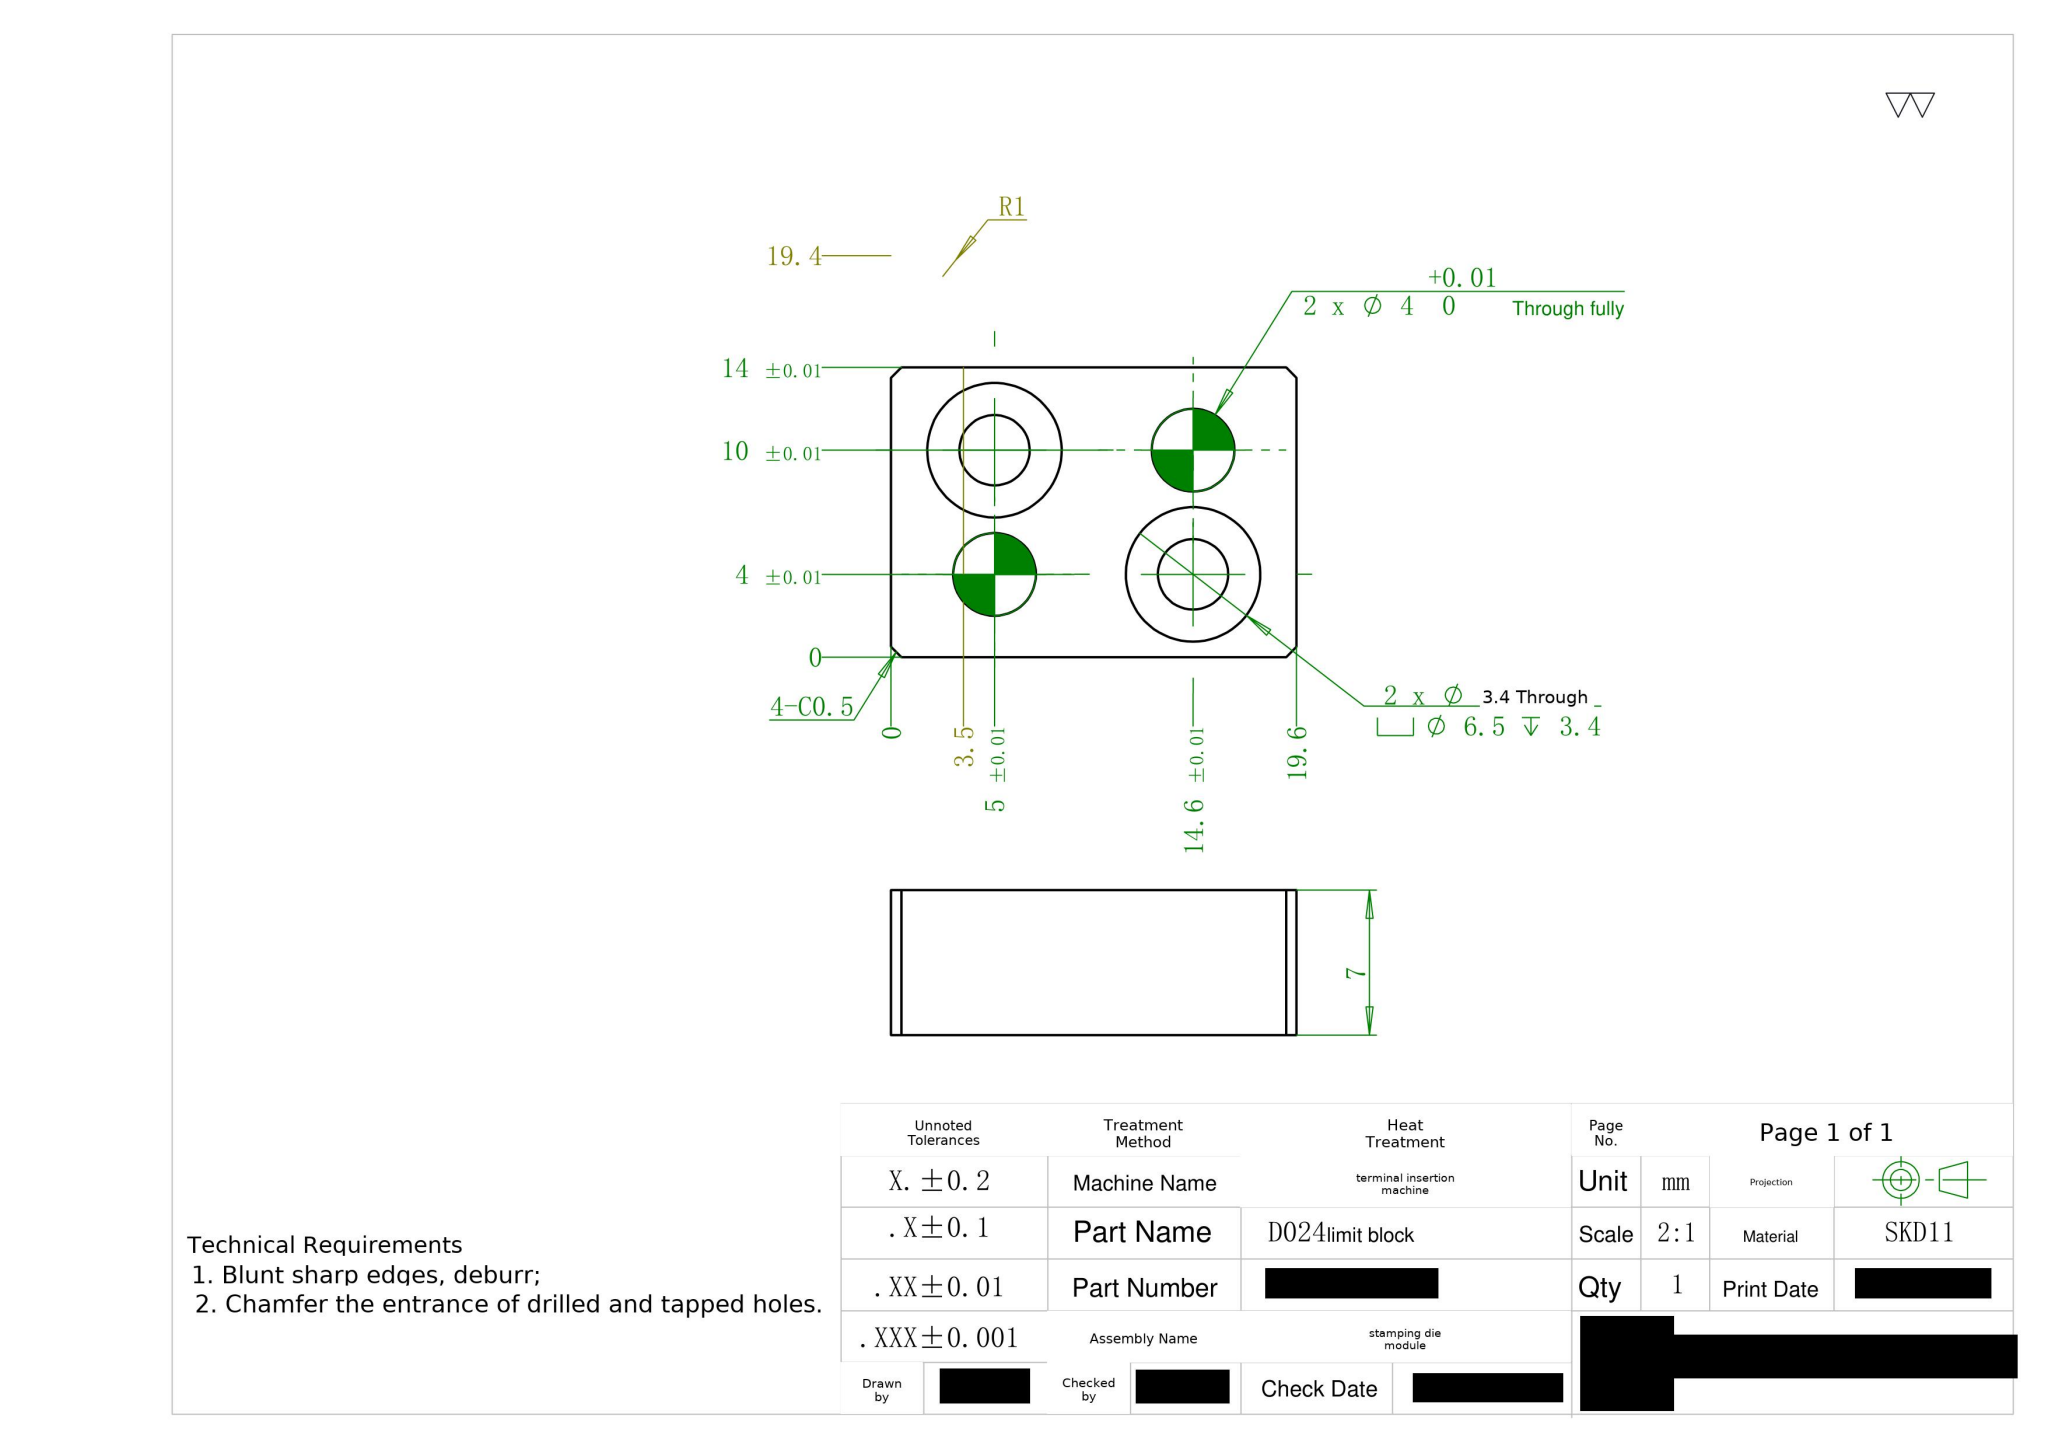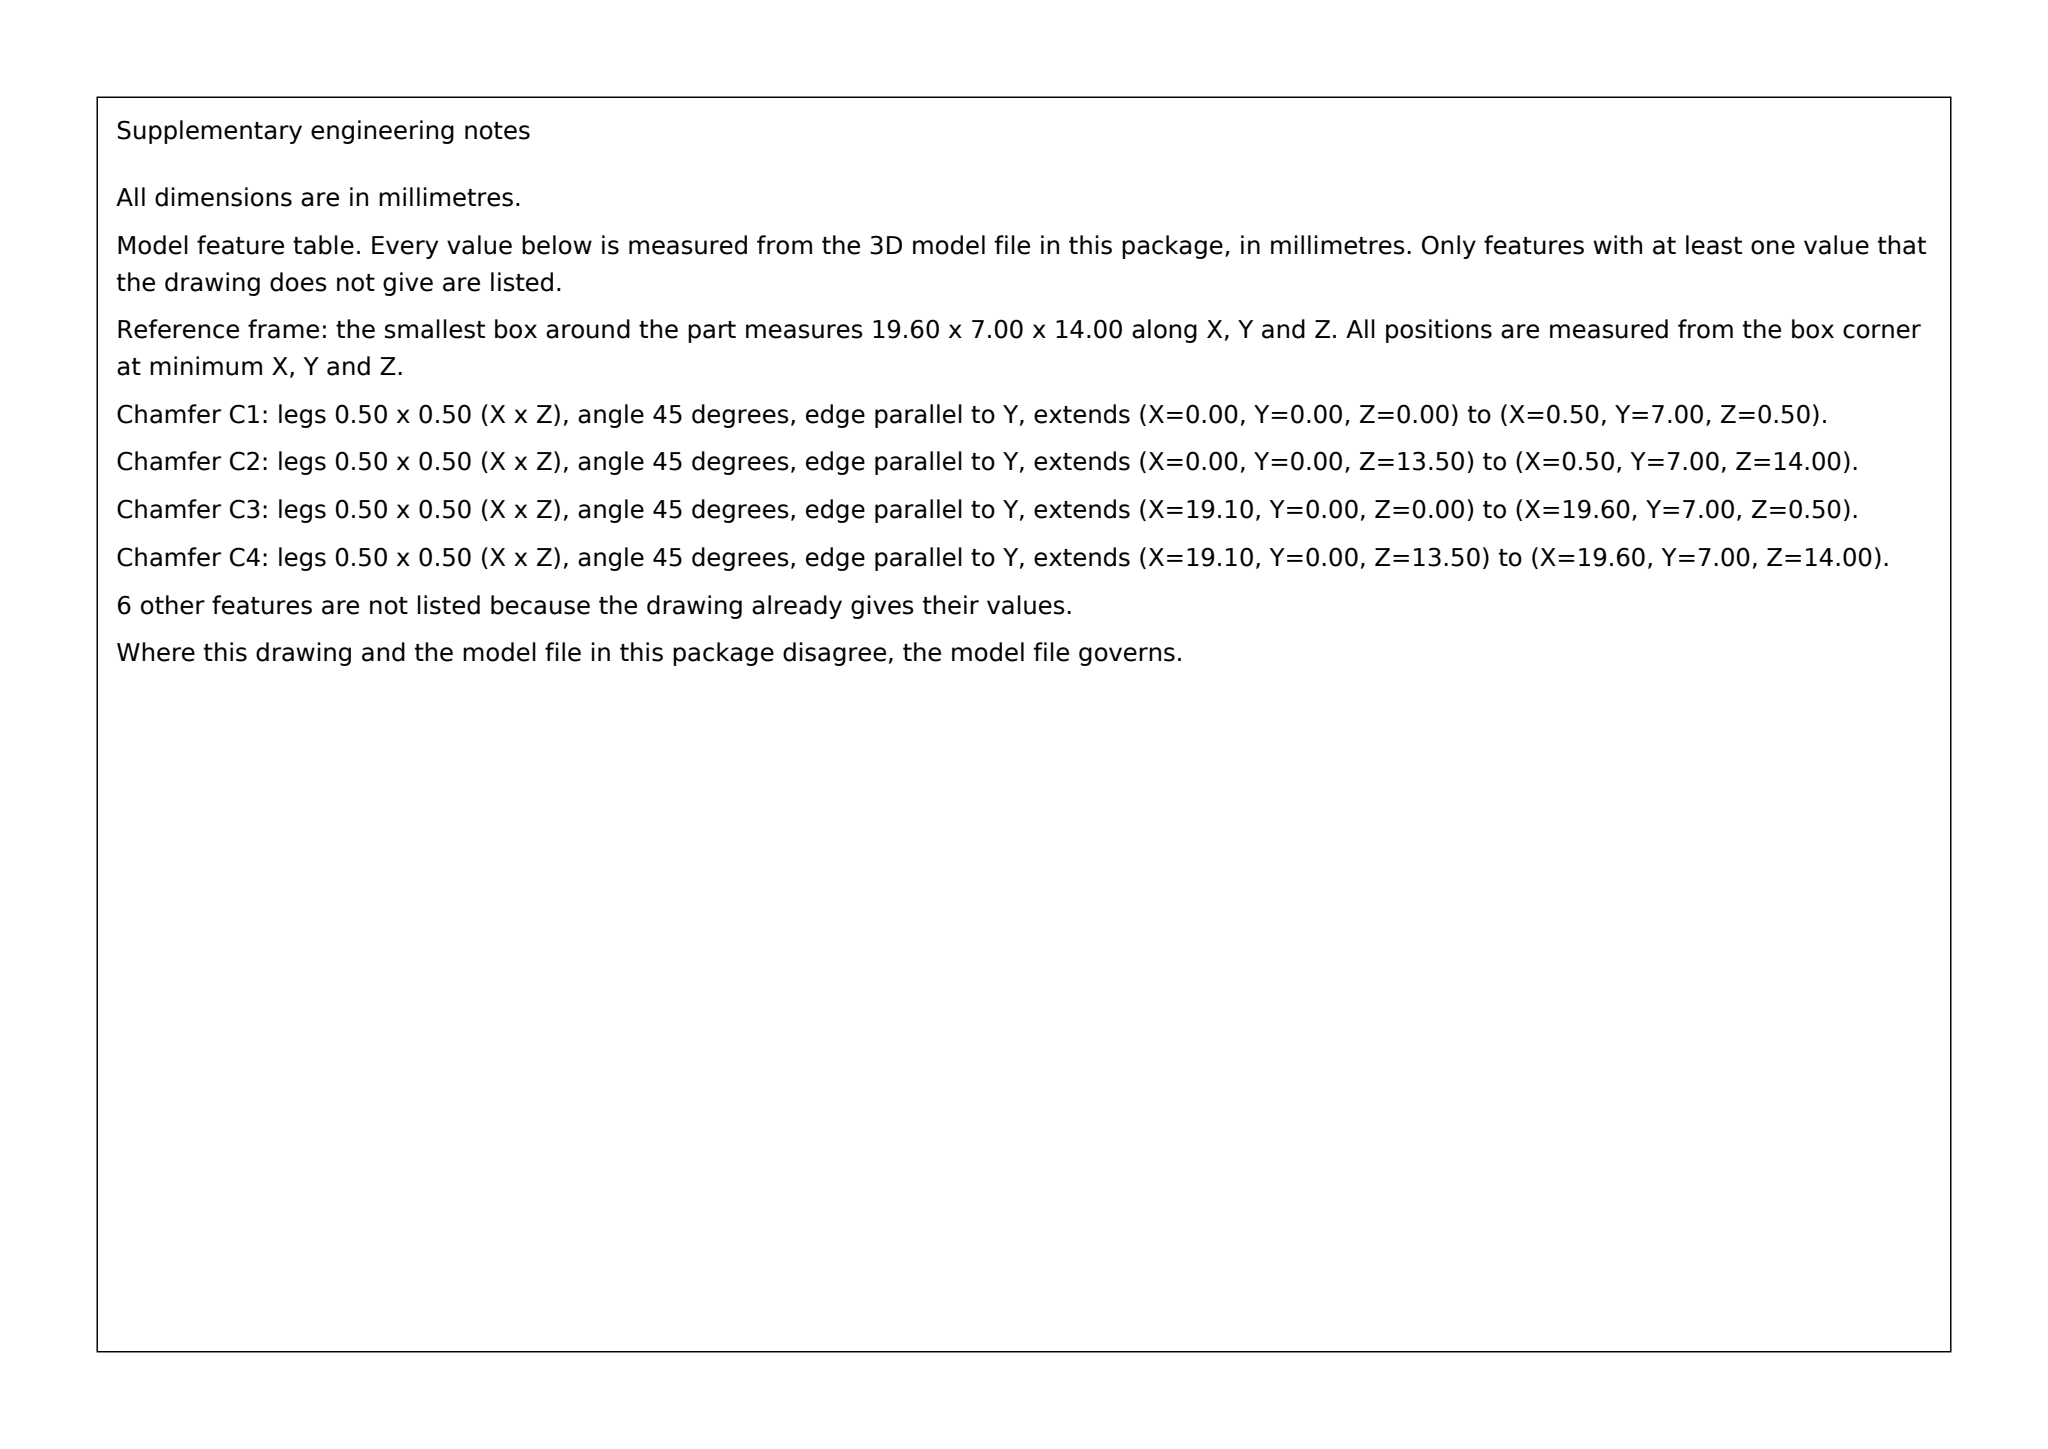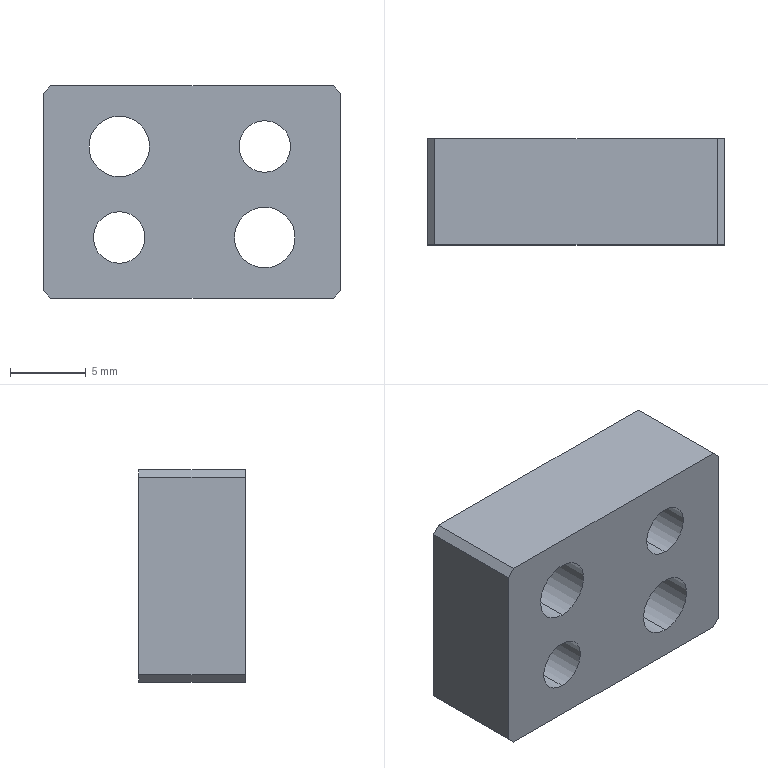Part | SolidWorks | mm | 1 solid | 24 faces | box 19.6 x 7 x 14 mm | volume 1450 mm3 | cylinder 12 | plane 12 | commonest cylinder face diameters 4 x4 6.5 x4 3.4 x4
build123d program:
from build123d import *

# Parameters (mm, degrees)
SKETCH1_W                                       = 19.6
SKETCH1_H                                       = 14
BOSS_EXTRUDE1_DEPTH                             = 7
M3_HEX_SOCKET_HEAD_CAP_SCREW_CBORE1_D           = 3.4
M3_HEX_SOCKET_HEAD_CAP_SCREW_CBORE1_CBORE_D     = 6.5
M3_HEX_SOCKET_HEAD_CAP_SCREW_CBORE1_CBORE_DEPTH = 3.4
F_4_0_4_DIAMETER_HOLE1_D                        = 4
CHAMFER1_SIZE                                   = 0.5


with BuildPart() as part:
    # Sketch1 → Boss-Extrude1 (new body)
    with BuildSketch(Plane(origin=(0, 0, 0), x_dir=(1, 0, 0), z_dir=(0, 1, 0))):
        Rectangle(SKETCH1_W, SKETCH1_H)
    extrude(amount=BOSS_EXTRUDE1_DEPTH)

    # M3 Hex Socket Head Cap Screw CBORE1 (through all)
    with Locations(Plane(origin=(0, 7, 0), x_dir=(1, 0, 0), z_dir=(0, 1, 0))):
        with Locations((4.8, -3), (-4.8, 3)):
            CounterBoreHole(M3_HEX_SOCKET_HEAD_CAP_SCREW_CBORE1_D / 2, M3_HEX_SOCKET_HEAD_CAP_SCREW_CBORE1_CBORE_D / 2, M3_HEX_SOCKET_HEAD_CAP_SCREW_CBORE1_CBORE_DEPTH)

    # 4.0 _4_ Diameter Hole1 (through all)
    with Locations(Plane(origin=(0, 7, 0), x_dir=(1, 0, 0), z_dir=(0, 1, 0))):
        with Locations((4.8, 3), (-4.8, -3)):
            Hole(F_4_0_4_DIAMETER_HOLE1_D / 2)

    # Chamfer1
    chamfer1_edges = [part.edges().sort_by_distance(p)[0] for p in [
        (9.8, 3.5, 7),
        (-9.8, 3.5, 7),
        (-9.8, 3.5, -7),
        (9.8, 3.5, -7),
    ]]
    chamfer(chamfer1_edges, length=CHAMFER1_SIZE)


solid = part.part
STEP:
#1=CARTESIAN_POINT('',(4.8,0.,-5.));
#2=VERTEX_POINT('',#1);
#3=CARTESIAN_POINT('',(4.8,0.,-1.));
#4=VERTEX_POINT('',#3);
#5=CARTESIAN_POINT('',(4.8,0.,-3.));
#6=DIRECTION('',(0.,1.,0.));
#7=DIRECTION('',(0.,0.,1.));
#8=AXIS2_PLACEMENT_3D('',#5,#6,#7);
#9=CIRCLE('',#8,2.);
#10=EDGE_CURVE('',#2,#4,#9,.T.);
#11=ORIENTED_EDGE('',*,*,#10,.F.);
#12=CARTESIAN_POINT('',(4.8,7.,-5.));
#13=VERTEX_POINT('',#12);
#14=CARTESIAN_POINT('',(4.8,7.,-5.));
#15=DIRECTION('',(0.,1.,0.));
#16=VECTOR('',#15,1000.);
#17=LINE('',#14,#16);
#18=EDGE_CURVE('',#2,#13,#17,.T.);
#19=ORIENTED_EDGE('',*,*,#18,.T.);
#20=CARTESIAN_POINT('',(4.8,7.,-1.));
#21=VERTEX_POINT('',#20);
#22=CARTESIAN_POINT('',(4.8,7.,-3.));
#23=DIRECTION('',(0.,1.,0.));
#24=DIRECTION('',(0.,0.,1.));
#25=AXIS2_PLACEMENT_3D('',#22,#23,#24);
#26=CIRCLE('',#25,2.);
#27=EDGE_CURVE('',#13,#21,#26,.T.);
#28=ORIENTED_EDGE('',*,*,#27,.T.);
#29=CARTESIAN_POINT('',(4.8,7.,-1.));
#30=DIRECTION('',(0.,1.,0.));
#31=VECTOR('',#30,1000.);
#32=LINE('',#29,#31);
#33=EDGE_CURVE('',#4,#21,#32,.T.);
#34=ORIENTED_EDGE('',*,*,#33,.F.);
#35=EDGE_LOOP('',(#11,#19,#28,#34));
#36=FACE_OUTER_BOUND('',#35,.T.);
#37=CARTESIAN_POINT('',(4.8,7.,-3.));
#38=DIRECTION('',(0.,1.,0.));
#39=DIRECTION('',(0.,0.,1.));
#40=AXIS2_PLACEMENT_3D('',#37,#38,#39);
#41=CYLINDRICAL_SURFACE('',#40,2.);
#42=ADVANCED_FACE('',(#36),#41,.F.);
#43=CARTESIAN_POINT('',(-4.8,0.,1.));
#44=VERTEX_POINT('',#43);
#45=CARTESIAN_POINT('',(-4.8,0.,5.));
#46=VERTEX_POINT('',#45);
#47=CARTESIAN_POINT('',(-4.8,0.,3.));
#48=DIRECTION('',(0.,1.,0.));
#49=DIRECTION('',(0.,0.,1.));
#50=AXIS2_PLACEMENT_3D('',#47,#48,#49);
#51=CIRCLE('',#50,2.);
#52=EDGE_CURVE('',#44,#46,#51,.T.);
#53=ORIENTED_EDGE('',*,*,#52,.F.);
#54=CARTESIAN_POINT('',(-4.8,7.,1.));
#55=VERTEX_POINT('',#54);
#56=CARTESIAN_POINT('',(-4.8,7.,1.));
#57=DIRECTION('',(0.,1.,0.));
#58=VECTOR('',#57,1000.);
#59=LINE('',#56,#58);
#60=EDGE_CURVE('',#44,#55,#59,.T.);
#61=ORIENTED_EDGE('',*,*,#60,.T.);
#62=CARTESIAN_POINT('',(-4.8,7.,5.));
#63=VERTEX_POINT('',#62);
#64=CARTESIAN_POINT('',(-4.8,7.,3.));
#65=DIRECTION('',(0.,1.,0.));
#66=DIRECTION('',(0.,0.,1.));
#67=AXIS2_PLACEMENT_3D('',#64,#65,#66);
#68=CIRCLE('',#67,2.);
#69=EDGE_CURVE('',#55,#63,#68,.T.);
#70=ORIENTED_EDGE('',*,*,#69,.T.);
#71=CARTESIAN_POINT('',(-4.8,7.,5.));
#72=DIRECTION('',(0.,1.,0.));
#73=VECTOR('',#72,1000.);
#74=LINE('',#71,#73);
#75=EDGE_CURVE('',#46,#63,#74,.T.);
#76=ORIENTED_EDGE('',*,*,#75,.F.);
#77=EDGE_LOOP('',(#53,#61,#70,#76));
#78=FACE_OUTER_BOUND('',#77,.T.);
#79=CARTESIAN_POINT('',(-4.8,7.,3.));
#80=DIRECTION('',(0.,1.,0.));
#81=DIRECTION('',(0.,0.,1.));
#82=AXIS2_PLACEMENT_3D('',#79,#80,#81);
#83=CYLINDRICAL_SURFACE('',#82,2.);
#84=ADVANCED_FACE('',(#78),#83,.F.);
#85=CARTESIAN_POINT('',(4.8,3.6,-0.25));
#86=VERTEX_POINT('',#85);
#87=CARTESIAN_POINT('',(4.8,3.6,6.25));
#88=VERTEX_POINT('',#87);
#89=CARTESIAN_POINT('',(4.8,3.6,3.));
#90=DIRECTION('',(0.,1.,0.));
#91=DIRECTION('',(0.,0.,1.));
#92=AXIS2_PLACEMENT_3D('',#89,#90,#91);
#93=CIRCLE('',#92,3.25);
#94=EDGE_CURVE('',#86,#88,#93,.T.);
#95=ORIENTED_EDGE('',*,*,#94,.F.);
#96=CARTESIAN_POINT('',(4.8,7.,-0.25));
#97=VERTEX_POINT('',#96);
#98=CARTESIAN_POINT('',(4.8,7.,-0.25));
#99=DIRECTION('',(0.,1.,0.));
#100=VECTOR('',#99,1000.);
#101=LINE('',#98,#100);
#102=EDGE_CURVE('',#86,#97,#101,.T.);
#103=ORIENTED_EDGE('',*,*,#102,.T.);
#104=CARTESIAN_POINT('',(4.8,7.,6.25));
#105=VERTEX_POINT('',#104);
#106=CARTESIAN_POINT('',(4.8,7.,3.));
#107=DIRECTION('',(0.,1.,0.));
#108=DIRECTION('',(0.,0.,1.));
#109=AXIS2_PLACEMENT_3D('',#106,#107,#108);
#110=CIRCLE('',#109,3.25);
#111=EDGE_CURVE('',#97,#105,#110,.T.);
#112=ORIENTED_EDGE('',*,*,#111,.T.);
#113=CARTESIAN_POINT('',(4.8,7.,6.25));
#114=DIRECTION('',(0.,1.,0.));
#115=VECTOR('',#114,1000.);
#116=LINE('',#113,#115);
#117=EDGE_CURVE('',#88,#105,#116,.T.);
#118=ORIENTED_EDGE('',*,*,#117,.F.);
#119=EDGE_LOOP('',(#95,#103,#112,#118));
#120=FACE_OUTER_BOUND('',#119,.T.);
#121=CARTESIAN_POINT('',(4.8,7.,3.));
#122=DIRECTION('',(0.,1.,0.));
#123=DIRECTION('',(0.,0.,1.));
#124=AXIS2_PLACEMENT_3D('',#121,#122,#123);
#125=CYLINDRICAL_SURFACE('',#124,3.25);
#126=ADVANCED_FACE('',(#120),#125,.F.);
#127=CARTESIAN_POINT('',(4.8,0.,1.3));
#128=VERTEX_POINT('',#127);
#129=CARTESIAN_POINT('',(4.8,0.,4.7));
#130=VERTEX_POINT('',#129);
#131=CARTESIAN_POINT('',(4.8,0.,3.));
#132=DIRECTION('',(0.,1.,0.));
#133=DIRECTION('',(0.,0.,1.));
#134=AXIS2_PLACEMENT_3D('',#131,#132,#133);
#135=CIRCLE('',#134,1.7);
#136=EDGE_CURVE('',#128,#130,#135,.T.);
#137=ORIENTED_EDGE('',*,*,#136,.F.);
#138=CARTESIAN_POINT('',(4.8,3.6,1.3));
#139=VERTEX_POINT('',#138);
#140=CARTESIAN_POINT('',(4.8,7.,1.3));
#141=DIRECTION('',(0.,1.,0.));
#142=VECTOR('',#141,1000.);
#143=LINE('',#140,#142);
#144=EDGE_CURVE('',#128,#139,#143,.T.);
#145=ORIENTED_EDGE('',*,*,#144,.T.);
#146=CARTESIAN_POINT('',(4.8,3.6,4.7));
#147=VERTEX_POINT('',#146);
#148=CARTESIAN_POINT('',(4.8,3.6,3.));
#149=DIRECTION('',(0.,1.,0.));
#150=DIRECTION('',(0.,0.,1.));
#151=AXIS2_PLACEMENT_3D('',#148,#149,#150);
#152=CIRCLE('',#151,1.7);
#153=EDGE_CURVE('',#139,#147,#152,.T.);
#154=ORIENTED_EDGE('',*,*,#153,.T.);
#155=CARTESIAN_POINT('',(4.8,7.,4.7));
#156=DIRECTION('',(0.,1.,0.));
#157=VECTOR('',#156,1000.);
#158=LINE('',#155,#157);
#159=EDGE_CURVE('',#130,#147,#158,.T.);
#160=ORIENTED_EDGE('',*,*,#159,.F.);
#161=EDGE_LOOP('',(#137,#145,#154,#160));
#162=FACE_OUTER_BOUND('',#161,.T.);
#163=CARTESIAN_POINT('',(4.8,7.,3.));
#164=DIRECTION('',(0.,1.,0.));
#165=DIRECTION('',(0.,0.,1.));
#166=AXIS2_PLACEMENT_3D('',#163,#164,#165);
#167=CYLINDRICAL_SURFACE('',#166,1.7);
#168=ADVANCED_FACE('',(#162),#167,.F.);
#169=CARTESIAN_POINT('',(-4.8,3.6,-6.25));
#170=VERTEX_POINT('',#169);
#171=CARTESIAN_POINT('',(-4.8,3.6,0.25));
#172=VERTEX_POINT('',#171);
#173=CARTESIAN_POINT('',(-4.8,3.6,-3.));
#174=DIRECTION('',(0.,1.,0.));
#175=DIRECTION('',(0.,0.,1.));
#176=AXIS2_PLACEMENT_3D('',#173,#174,#175);
#177=CIRCLE('',#176,3.25);
#178=EDGE_CURVE('',#170,#172,#177,.T.);
#179=ORIENTED_EDGE('',*,*,#178,.F.);
#180=CARTESIAN_POINT('',(-4.8,7.,-6.25));
#181=VERTEX_POINT('',#180);
#182=CARTESIAN_POINT('',(-4.8,7.,-6.25));
#183=DIRECTION('',(0.,1.,0.));
#184=VECTOR('',#183,1000.);
#185=LINE('',#182,#184);
#186=EDGE_CURVE('',#170,#181,#185,.T.);
#187=ORIENTED_EDGE('',*,*,#186,.T.);
#188=CARTESIAN_POINT('',(-4.8,7.,0.25));
#189=VERTEX_POINT('',#188);
#190=CARTESIAN_POINT('',(-4.8,7.,-3.));
#191=DIRECTION('',(0.,1.,0.));
#192=DIRECTION('',(0.,0.,1.));
#193=AXIS2_PLACEMENT_3D('',#190,#191,#192);
#194=CIRCLE('',#193,3.25);
#195=EDGE_CURVE('',#181,#189,#194,.T.);
#196=ORIENTED_EDGE('',*,*,#195,.T.);
#197=CARTESIAN_POINT('',(-4.8,7.,0.25));
#198=DIRECTION('',(0.,1.,0.));
#199=VECTOR('',#198,1000.);
#200=LINE('',#197,#199);
#201=EDGE_CURVE('',#172,#189,#200,.T.);
#202=ORIENTED_EDGE('',*,*,#201,.F.);
#203=EDGE_LOOP('',(#179,#187,#196,#202));
#204=FACE_OUTER_BOUND('',#203,.T.);
#205=CARTESIAN_POINT('',(-4.8,7.,-3.));
#206=DIRECTION('',(0.,1.,0.));
#207=DIRECTION('',(0.,0.,1.));
#208=AXIS2_PLACEMENT_3D('',#205,#206,#207);
#209=CYLINDRICAL_SURFACE('',#208,3.25);
#210=ADVANCED_FACE('',(#204),#209,.F.);
#211=CARTESIAN_POINT('',(-4.8,0.,-4.7));
#212=VERTEX_POINT('',#211);
#213=CARTESIAN_POINT('',(-4.8,0.,-1.3));
#214=VERTEX_POINT('',#213);
#215=CARTESIAN_POINT('',(-4.8,0.,-3.));
#216=DIRECTION('',(0.,1.,0.));
#217=DIRECTION('',(0.,0.,1.));
#218=AXIS2_PLACEMENT_3D('',#215,#216,#217);
#219=CIRCLE('',#218,1.7);
#220=EDGE_CURVE('',#212,#214,#219,.T.);
#221=ORIENTED_EDGE('',*,*,#220,.F.);
#222=CARTESIAN_POINT('',(-4.8,3.6,-4.7));
#223=VERTEX_POINT('',#222);
#224=CARTESIAN_POINT('',(-4.8,7.,-4.7));
#225=DIRECTION('',(0.,1.,0.));
#226=VECTOR('',#225,1000.);
#227=LINE('',#224,#226);
#228=EDGE_CURVE('',#212,#223,#227,.T.);
#229=ORIENTED_EDGE('',*,*,#228,.T.);
#230=CARTESIAN_POINT('',(-4.8,3.6,-1.3));
#231=VERTEX_POINT('',#230);
#232=CARTESIAN_POINT('',(-4.8,3.6,-3.));
#233=DIRECTION('',(0.,1.,0.));
#234=DIRECTION('',(0.,0.,1.));
#235=AXIS2_PLACEMENT_3D('',#232,#233,#234);
#236=CIRCLE('',#235,1.7);
#237=EDGE_CURVE('',#223,#231,#236,.T.);
#238=ORIENTED_EDGE('',*,*,#237,.T.);
#239=CARTESIAN_POINT('',(-4.8,7.,-1.3));
#240=DIRECTION('',(0.,1.,0.));
#241=VECTOR('',#240,1000.);
#242=LINE('',#239,#241);
#243=EDGE_CURVE('',#214,#231,#242,.T.);
#244=ORIENTED_EDGE('',*,*,#243,.F.);
#245=EDGE_LOOP('',(#221,#229,#238,#244));
#246=FACE_OUTER_BOUND('',#245,.T.);
#247=CARTESIAN_POINT('',(-4.8,7.,-3.));
#248=DIRECTION('',(0.,1.,0.));
#249=DIRECTION('',(0.,0.,1.));
#250=AXIS2_PLACEMENT_3D('',#247,#248,#249);
#251=CYLINDRICAL_SURFACE('',#250,1.7);
#252=ADVANCED_FACE('',(#246),#251,.F.);
#253=CARTESIAN_POINT('',(9.8,0.,6.5));
#254=VERTEX_POINT('',#253);
#255=CARTESIAN_POINT('',(9.8,0.,-6.5));
#256=VERTEX_POINT('',#255);
#257=CARTESIAN_POINT('',(9.8,0.,-7.));
#258=DIRECTION('',(-0.,0.,-1.));
#259=VECTOR('',#258,1000.);
#260=LINE('',#257,#259);
#261=EDGE_CURVE('',#254,#256,#260,.T.);
#262=ORIENTED_EDGE('',*,*,#261,.T.);
#263=CARTESIAN_POINT('',(9.8,7.,-6.5));
#264=VERTEX_POINT('',#263);
#265=CARTESIAN_POINT('',(9.8,7.,-6.5));
#266=DIRECTION('',(0.,1.,0.));
#267=VECTOR('',#266,1000.);
#268=LINE('',#265,#267);
#269=EDGE_CURVE('',#256,#264,#268,.T.);
#270=ORIENTED_EDGE('',*,*,#269,.T.);
#271=CARTESIAN_POINT('',(9.8,7.,6.5));
#272=VERTEX_POINT('',#271);
#273=CARTESIAN_POINT('',(9.8,7.,-7.));
#274=DIRECTION('',(-0.,0.,-1.));
#275=VECTOR('',#274,1000.);
#276=LINE('',#273,#275);
#277=EDGE_CURVE('',#272,#264,#276,.T.);
#278=ORIENTED_EDGE('',*,*,#277,.F.);
#279=CARTESIAN_POINT('',(9.8,7.,6.5));
#280=DIRECTION('',(0.,-1.,0.));
#281=VECTOR('',#280,1000.);
#282=LINE('',#279,#281);
#283=EDGE_CURVE('',#272,#254,#282,.T.);
#284=ORIENTED_EDGE('',*,*,#283,.T.);
#285=EDGE_LOOP('',(#262,#270,#278,#284));
#286=FACE_OUTER_BOUND('',#285,.T.);
#287=CARTESIAN_POINT('',(9.8,7.,-7.));
#288=DIRECTION('',(-1.,0.,0.));
#289=DIRECTION('',(0.,0.,1.));
#290=AXIS2_PLACEMENT_3D('',#287,#288,#289);
#291=PLANE('',#290);
#292=ADVANCED_FACE('',(#286),#291,.F.);
#293=CARTESIAN_POINT('',(9.3,0.,-7.));
#294=VERTEX_POINT('',#293);
#295=CARTESIAN_POINT('',(-9.3,0.,-7.));
#296=VERTEX_POINT('',#295);
#297=CARTESIAN_POINT('',(-9.8,0.,-7.));
#298=DIRECTION('',(-1.,0.,0.));
#299=VECTOR('',#298,1000.);
#300=LINE('',#297,#299);
#301=EDGE_CURVE('',#294,#296,#300,.T.);
#302=ORIENTED_EDGE('',*,*,#301,.T.);
#303=CARTESIAN_POINT('',(-9.3,7.,-7.));
#304=VERTEX_POINT('',#303);
#305=CARTESIAN_POINT('',(-9.3,7.,-7.));
#306=DIRECTION('',(0.,1.,0.));
#307=VECTOR('',#306,1000.);
#308=LINE('',#305,#307);
#309=EDGE_CURVE('',#296,#304,#308,.T.);
#310=ORIENTED_EDGE('',*,*,#309,.T.);
#311=CARTESIAN_POINT('',(9.3,7.,-7.));
#312=VERTEX_POINT('',#311);
#313=CARTESIAN_POINT('',(-9.8,7.,-7.));
#314=DIRECTION('',(-1.,0.,0.));
#315=VECTOR('',#314,1000.);
#316=LINE('',#313,#315);
#317=EDGE_CURVE('',#312,#304,#316,.T.);
#318=ORIENTED_EDGE('',*,*,#317,.F.);
#319=CARTESIAN_POINT('',(9.3,7.,-7.));
#320=DIRECTION('',(0.,-1.,0.));
#321=VECTOR('',#320,1000.);
#322=LINE('',#319,#321);
#323=EDGE_CURVE('',#312,#294,#322,.T.);
#324=ORIENTED_EDGE('',*,*,#323,.T.);
#325=EDGE_LOOP('',(#302,#310,#318,#324));
#326=FACE_OUTER_BOUND('',#325,.T.);
#327=CARTESIAN_POINT('',(-9.8,7.,-7.));
#328=DIRECTION('',(0.,0.,1.));
#329=DIRECTION('',(1.,0.,0.));
#330=AXIS2_PLACEMENT_3D('',#327,#328,#329);
#331=PLANE('',#330);
#332=ADVANCED_FACE('',(#326),#331,.F.);
#333=CARTESIAN_POINT('',(-9.8,7.,-6.5));
#334=VERTEX_POINT('',#333);
#335=CARTESIAN_POINT('',(-9.8,7.,6.5));
#336=VERTEX_POINT('',#335);
#337=CARTESIAN_POINT('',(-9.8,7.,-7.));
#338=DIRECTION('',(0.,0.,1.));
#339=VECTOR('',#338,1000.);
#340=LINE('',#337,#339);
#341=EDGE_CURVE('',#334,#336,#340,.T.);
#342=ORIENTED_EDGE('',*,*,#341,.F.);
#343=CARTESIAN_POINT('',(-9.8,0.,-6.5));
#344=VERTEX_POINT('',#343);
#345=CARTESIAN_POINT('',(-9.8,7.,-6.5));
#346=DIRECTION('',(0.,-1.,0.));
#347=VECTOR('',#346,1000.);
#348=LINE('',#345,#347);
#349=EDGE_CURVE('',#334,#344,#348,.T.);
#350=ORIENTED_EDGE('',*,*,#349,.T.);
#351=CARTESIAN_POINT('',(-9.8,0.,6.5));
#352=VERTEX_POINT('',#351);
#353=CARTESIAN_POINT('',(-9.8,0.,-7.));
#354=DIRECTION('',(0.,0.,1.));
#355=VECTOR('',#354,1000.);
#356=LINE('',#353,#355);
#357=EDGE_CURVE('',#344,#352,#356,.T.);
#358=ORIENTED_EDGE('',*,*,#357,.T.);
#359=CARTESIAN_POINT('',(-9.8,7.,6.5));
#360=DIRECTION('',(0.,1.,0.));
#361=VECTOR('',#360,1000.);
#362=LINE('',#359,#361);
#363=EDGE_CURVE('',#352,#336,#362,.T.);
#364=ORIENTED_EDGE('',*,*,#363,.T.);
#365=EDGE_LOOP('',(#342,#350,#358,#364));
#366=FACE_OUTER_BOUND('',#365,.T.);
#367=CARTESIAN_POINT('',(-9.8,7.,-7.));
#368=DIRECTION('',(1.,0.,-0.));
#369=DIRECTION('',(-0.,0.,-1.));
#370=AXIS2_PLACEMENT_3D('',#367,#368,#369);
#371=PLANE('',#370);
#372=ADVANCED_FACE('',(#366),#371,.F.);
#373=CARTESIAN_POINT('',(-9.3,7.,7.));
#374=VERTEX_POINT('',#373);
#375=CARTESIAN_POINT('',(9.3,7.,7.));
#376=VERTEX_POINT('',#375);
#377=CARTESIAN_POINT('',(-9.8,7.,7.));
#378=DIRECTION('',(1.,0.,0.));
#379=VECTOR('',#378,1000.);
#380=LINE('',#377,#379);
#381=EDGE_CURVE('',#374,#376,#380,.T.);
#382=ORIENTED_EDGE('',*,*,#381,.F.);
#383=CARTESIAN_POINT('',(-9.3,0.,7.));
#384=VERTEX_POINT('',#383);
#385=CARTESIAN_POINT('',(-9.3,7.,7.));
#386=DIRECTION('',(0.,-1.,0.));
#387=VECTOR('',#386,1000.);
#388=LINE('',#385,#387);
#389=EDGE_CURVE('',#374,#384,#388,.T.);
#390=ORIENTED_EDGE('',*,*,#389,.T.);
#391=CARTESIAN_POINT('',(9.3,0.,7.));
#392=VERTEX_POINT('',#391);
#393=CARTESIAN_POINT('',(-9.8,0.,7.));
#394=DIRECTION('',(1.,0.,0.));
#395=VECTOR('',#394,1000.);
#396=LINE('',#393,#395);
#397=EDGE_CURVE('',#384,#392,#396,.T.);
#398=ORIENTED_EDGE('',*,*,#397,.T.);
#399=CARTESIAN_POINT('',(9.3,7.,7.));
#400=DIRECTION('',(0.,1.,0.));
#401=VECTOR('',#400,1000.);
#402=LINE('',#399,#401);
#403=EDGE_CURVE('',#392,#376,#402,.T.);
#404=ORIENTED_EDGE('',*,*,#403,.T.);
#405=EDGE_LOOP('',(#382,#390,#398,#404));
#406=FACE_OUTER_BOUND('',#405,.T.);
#407=CARTESIAN_POINT('',(-9.8,7.,7.));
#408=DIRECTION('',(0.,0.,-1.));
#409=DIRECTION('',(-1.,0.,0.));
#410=AXIS2_PLACEMENT_3D('',#407,#408,#409);
#411=PLANE('',#410);
#412=ADVANCED_FACE('',(#406),#411,.F.);
#413=CARTESIAN_POINT('',(4.8,7.,-3.));
#414=DIRECTION('',(0.,1.,0.));
#415=DIRECTION('',(0.,0.,1.));
#416=AXIS2_PLACEMENT_3D('',#413,#414,#415);
#417=CIRCLE('',#416,2.);
#418=EDGE_CURVE('',#21,#13,#417,.T.);
#419=ORIENTED_EDGE('',*,*,#418,.F.);
#420=ORIENTED_EDGE('',*,*,#27,.F.);
#421=EDGE_LOOP('',(#419,#420));
#422=FACE_BOUND('',#421,.T.);
#423=CARTESIAN_POINT('',(-4.8,7.,3.));
#424=DIRECTION('',(0.,1.,0.));
#425=DIRECTION('',(0.,0.,1.));
#426=AXIS2_PLACEMENT_3D('',#423,#424,#425);
#427=CIRCLE('',#426,2.);
#428=EDGE_CURVE('',#63,#55,#427,.T.);
#429=ORIENTED_EDGE('',*,*,#428,.F.);
#430=ORIENTED_EDGE('',*,*,#69,.F.);
#431=EDGE_LOOP('',(#429,#430));
#432=FACE_BOUND('',#431,.T.);
#433=CARTESIAN_POINT('',(4.8,7.,3.));
#434=DIRECTION('',(0.,1.,0.));
#435=DIRECTION('',(0.,0.,1.));
#436=AXIS2_PLACEMENT_3D('',#433,#434,#435);
#437=CIRCLE('',#436,3.25);
#438=EDGE_CURVE('',#105,#97,#437,.T.);
#439=ORIENTED_EDGE('',*,*,#438,.F.);
#440=ORIENTED_EDGE('',*,*,#111,.F.);
#441=EDGE_LOOP('',(#439,#440));
#442=FACE_BOUND('',#441,.T.);
#443=CARTESIAN_POINT('',(-4.8,7.,-3.));
#444=DIRECTION('',(0.,1.,0.));
#445=DIRECTION('',(0.,0.,1.));
#446=AXIS2_PLACEMENT_3D('',#443,#444,#445);
#447=CIRCLE('',#446,3.25);
#448=EDGE_CURVE('',#189,#181,#447,.T.);
#449=ORIENTED_EDGE('',*,*,#448,.F.);
#450=ORIENTED_EDGE('',*,*,#195,.F.);
#451=EDGE_LOOP('',(#449,#450));
#452=FACE_BOUND('',#451,.T.);
#453=ORIENTED_EDGE('',*,*,#317,.T.);
#454=CARTESIAN_POINT('',(-8.15,7.,-8.15));
#455=DIRECTION('',(-0.7071,0.,0.7071));
#456=VECTOR('',#455,1000.);
#457=LINE('',#454,#456);
#458=EDGE_CURVE('',#304,#334,#457,.T.);
#459=ORIENTED_EDGE('',*,*,#458,.T.);
#460=ORIENTED_EDGE('',*,*,#341,.T.);
#461=CARTESIAN_POINT('',(-8.15,7.,8.15));
#462=DIRECTION('',(0.7071,0.,0.7071));
#463=VECTOR('',#462,1000.);
#464=LINE('',#461,#463);
#465=EDGE_CURVE('',#336,#374,#464,.T.);
#466=ORIENTED_EDGE('',*,*,#465,.T.);
#467=ORIENTED_EDGE('',*,*,#381,.T.);
#468=CARTESIAN_POINT('',(8.15,7.,8.15));
#469=DIRECTION('',(0.7071,0.,-0.7071));
#470=VECTOR('',#469,1000.);
#471=LINE('',#468,#470);
#472=EDGE_CURVE('',#376,#272,#471,.T.);
#473=ORIENTED_EDGE('',*,*,#472,.T.);
#474=ORIENTED_EDGE('',*,*,#277,.T.);
#475=CARTESIAN_POINT('',(8.15,7.,-8.15));
#476=DIRECTION('',(-0.7071,0.,-0.7071));
#477=VECTOR('',#476,1000.);
#478=LINE('',#475,#477);
#479=EDGE_CURVE('',#264,#312,#478,.T.);
#480=ORIENTED_EDGE('',*,*,#479,.T.);
#481=EDGE_LOOP('',(#453,#459,#460,#466,#467,#473,#474,#480));
#482=FACE_OUTER_BOUND('',#481,.T.);
#483=CARTESIAN_POINT('',(0.,7.,0.));
#484=DIRECTION('',(0.,1.,0.));
#485=DIRECTION('',(0.,0.,1.));
#486=AXIS2_PLACEMENT_3D('',#483,#484,#485);
#487=PLANE('',#486);
#488=ADVANCED_FACE('',(#422,#432,#442,#452,#482),#487,.T.);
#489=CARTESIAN_POINT('',(4.8,0.,-3.));
#490=DIRECTION('',(0.,1.,0.));
#491=DIRECTION('',(0.,0.,1.));
#492=AXIS2_PLACEMENT_3D('',#489,#490,#491);
#493=CIRCLE('',#492,2.);
#494=EDGE_CURVE('',#4,#2,#493,.T.);
#495=ORIENTED_EDGE('',*,*,#494,.T.);
#496=ORIENTED_EDGE('',*,*,#10,.T.);
#497=EDGE_LOOP('',(#495,#496));
#498=FACE_BOUND('',#497,.T.);
#499=CARTESIAN_POINT('',(-4.8,0.,3.));
#500=DIRECTION('',(0.,1.,0.));
#501=DIRECTION('',(0.,0.,1.));
#502=AXIS2_PLACEMENT_3D('',#499,#500,#501);
#503=CIRCLE('',#502,2.);
#504=EDGE_CURVE('',#46,#44,#503,.T.);
#505=ORIENTED_EDGE('',*,*,#504,.T.);
#506=ORIENTED_EDGE('',*,*,#52,.T.);
#507=EDGE_LOOP('',(#505,#506));
#508=FACE_BOUND('',#507,.T.);
#509=CARTESIAN_POINT('',(4.8,0.,3.));
#510=DIRECTION('',(0.,1.,0.));
#511=DIRECTION('',(0.,0.,1.));
#512=AXIS2_PLACEMENT_3D('',#509,#510,#511);
#513=CIRCLE('',#512,1.7);
#514=EDGE_CURVE('',#130,#128,#513,.T.);
#515=ORIENTED_EDGE('',*,*,#514,.T.);
#516=ORIENTED_EDGE('',*,*,#136,.T.);
#517=EDGE_LOOP('',(#515,#516));
#518=FACE_BOUND('',#517,.T.);
#519=CARTESIAN_POINT('',(-4.8,0.,-3.));
#520=DIRECTION('',(0.,1.,0.));
#521=DIRECTION('',(0.,0.,1.));
#522=AXIS2_PLACEMENT_3D('',#519,#520,#521);
#523=CIRCLE('',#522,1.7);
#524=EDGE_CURVE('',#214,#212,#523,.T.);
#525=ORIENTED_EDGE('',*,*,#524,.T.);
#526=ORIENTED_EDGE('',*,*,#220,.T.);
#527=EDGE_LOOP('',(#525,#526));
#528=FACE_BOUND('',#527,.T.);
#529=ORIENTED_EDGE('',*,*,#357,.F.);
#530=CARTESIAN_POINT('',(-9.8,0.,-6.5));
#531=DIRECTION('',(0.7071,0.,-0.7071));
#532=VECTOR('',#531,1000.);
#533=LINE('',#530,#532);
#534=EDGE_CURVE('',#344,#296,#533,.T.);
#535=ORIENTED_EDGE('',*,*,#534,.T.);
#536=ORIENTED_EDGE('',*,*,#301,.F.);
#537=CARTESIAN_POINT('',(9.3,0.,-7.));
#538=DIRECTION('',(0.7071,0.,0.7071));
#539=VECTOR('',#538,1000.);
#540=LINE('',#537,#539);
#541=EDGE_CURVE('',#294,#256,#540,.T.);
#542=ORIENTED_EDGE('',*,*,#541,.T.);
#543=ORIENTED_EDGE('',*,*,#261,.F.);
#544=CARTESIAN_POINT('',(9.8,0.,6.5));
#545=DIRECTION('',(-0.7071,0.,0.7071));
#546=VECTOR('',#545,1000.);
#547=LINE('',#544,#546);
#548=EDGE_CURVE('',#254,#392,#547,.T.);
#549=ORIENTED_EDGE('',*,*,#548,.T.);
#550=ORIENTED_EDGE('',*,*,#397,.F.);
#551=CARTESIAN_POINT('',(-9.3,0.,7.));
#552=DIRECTION('',(-0.7071,0.,-0.7071));
#553=VECTOR('',#552,1000.);
#554=LINE('',#551,#553);
#555=EDGE_CURVE('',#384,#352,#554,.T.);
#556=ORIENTED_EDGE('',*,*,#555,.T.);
#557=EDGE_LOOP('',(#529,#535,#536,#542,#543,#549,#550,#556));
#558=FACE_OUTER_BOUND('',#557,.T.);
#559=CARTESIAN_POINT('',(0.,0.,0.));
#560=DIRECTION('',(0.,1.,0.));
#561=DIRECTION('',(0.,0.,1.));
#562=AXIS2_PLACEMENT_3D('',#559,#560,#561);
#563=PLANE('',#562);
#564=ADVANCED_FACE('',(#498,#508,#518,#528,#558),#563,.F.);
#565=ORIENTED_EDGE('',*,*,#228,.F.);
#566=ORIENTED_EDGE('',*,*,#524,.F.);
#567=ORIENTED_EDGE('',*,*,#243,.T.);
#568=CARTESIAN_POINT('',(-4.8,3.6,-3.));
#569=DIRECTION('',(0.,1.,0.));
#570=DIRECTION('',(0.,0.,1.));
#571=AXIS2_PLACEMENT_3D('',#568,#569,#570);
#572=CIRCLE('',#571,1.7);
#573=EDGE_CURVE('',#231,#223,#572,.T.);
#574=ORIENTED_EDGE('',*,*,#573,.T.);
#575=EDGE_LOOP('',(#565,#566,#567,#574));
#576=FACE_OUTER_BOUND('',#575,.T.);
#577=CARTESIAN_POINT('',(-4.8,7.,-3.));
#578=DIRECTION('',(0.,1.,0.));
#579=DIRECTION('',(0.,0.,1.));
#580=AXIS2_PLACEMENT_3D('',#577,#578,#579);
#581=CYLINDRICAL_SURFACE('',#580,1.7);
#582=ADVANCED_FACE('',(#576),#581,.F.);
#583=ORIENTED_EDGE('',*,*,#573,.F.);
#584=ORIENTED_EDGE('',*,*,#237,.F.);
#585=EDGE_LOOP('',(#583,#584));
#586=FACE_BOUND('',#585,.T.);
#587=CARTESIAN_POINT('',(-4.8,3.6,-3.));
#588=DIRECTION('',(0.,1.,0.));
#589=DIRECTION('',(0.,0.,1.));
#590=AXIS2_PLACEMENT_3D('',#587,#588,#589);
#591=CIRCLE('',#590,3.25);
#592=EDGE_CURVE('',#172,#170,#591,.T.);
#593=ORIENTED_EDGE('',*,*,#592,.T.);
#594=ORIENTED_EDGE('',*,*,#178,.T.);
#595=EDGE_LOOP('',(#593,#594));
#596=FACE_OUTER_BOUND('',#595,.T.);
#597=CARTESIAN_POINT('',(-3.1,3.6,-3.));
#598=DIRECTION('',(0.,-1.,0.));
#599=DIRECTION('',(0.,0.,-1.));
#600=AXIS2_PLACEMENT_3D('',#597,#598,#599);
#601=PLANE('',#600);
#602=ADVANCED_FACE('',(#586,#596),#601,.F.);
#603=ORIENTED_EDGE('',*,*,#186,.F.);
#604=ORIENTED_EDGE('',*,*,#592,.F.);
#605=ORIENTED_EDGE('',*,*,#201,.T.);
#606=ORIENTED_EDGE('',*,*,#448,.T.);
#607=EDGE_LOOP('',(#603,#604,#605,#606));
#608=FACE_OUTER_BOUND('',#607,.T.);
#609=CARTESIAN_POINT('',(-4.8,7.,-3.));
#610=DIRECTION('',(0.,1.,0.));
#611=DIRECTION('',(0.,0.,1.));
#612=AXIS2_PLACEMENT_3D('',#609,#610,#611);
#613=CYLINDRICAL_SURFACE('',#612,3.25);
#614=ADVANCED_FACE('',(#608),#613,.F.);
#615=ORIENTED_EDGE('',*,*,#144,.F.);
#616=ORIENTED_EDGE('',*,*,#514,.F.);
#617=ORIENTED_EDGE('',*,*,#159,.T.);
#618=CARTESIAN_POINT('',(4.8,3.6,3.));
#619=DIRECTION('',(0.,1.,0.));
#620=DIRECTION('',(0.,0.,1.));
#621=AXIS2_PLACEMENT_3D('',#618,#619,#620);
#622=CIRCLE('',#621,1.7);
#623=EDGE_CURVE('',#147,#139,#622,.T.);
#624=ORIENTED_EDGE('',*,*,#623,.T.);
#625=EDGE_LOOP('',(#615,#616,#617,#624));
#626=FACE_OUTER_BOUND('',#625,.T.);
#627=CARTESIAN_POINT('',(4.8,7.,3.));
#628=DIRECTION('',(0.,1.,0.));
#629=DIRECTION('',(0.,0.,1.));
#630=AXIS2_PLACEMENT_3D('',#627,#628,#629);
#631=CYLINDRICAL_SURFACE('',#630,1.7);
#632=ADVANCED_FACE('',(#626),#631,.F.);
#633=ORIENTED_EDGE('',*,*,#623,.F.);
#634=ORIENTED_EDGE('',*,*,#153,.F.);
#635=EDGE_LOOP('',(#633,#634));
#636=FACE_BOUND('',#635,.T.);
#637=CARTESIAN_POINT('',(4.8,3.6,3.));
#638=DIRECTION('',(0.,1.,0.));
#639=DIRECTION('',(0.,0.,1.));
#640=AXIS2_PLACEMENT_3D('',#637,#638,#639);
#641=CIRCLE('',#640,3.25);
#642=EDGE_CURVE('',#88,#86,#641,.T.);
#643=ORIENTED_EDGE('',*,*,#642,.T.);
#644=ORIENTED_EDGE('',*,*,#94,.T.);
#645=EDGE_LOOP('',(#643,#644));
#646=FACE_OUTER_BOUND('',#645,.T.);
#647=CARTESIAN_POINT('',(6.5,3.6,3.));
#648=DIRECTION('',(0.,-1.,0.));
#649=DIRECTION('',(0.,0.,-1.));
#650=AXIS2_PLACEMENT_3D('',#647,#648,#649);
#651=PLANE('',#650);
#652=ADVANCED_FACE('',(#636,#646),#651,.F.);
#653=ORIENTED_EDGE('',*,*,#102,.F.);
#654=ORIENTED_EDGE('',*,*,#642,.F.);
#655=ORIENTED_EDGE('',*,*,#117,.T.);
#656=ORIENTED_EDGE('',*,*,#438,.T.);
#657=EDGE_LOOP('',(#653,#654,#655,#656));
#658=FACE_OUTER_BOUND('',#657,.T.);
#659=CARTESIAN_POINT('',(4.8,7.,3.));
#660=DIRECTION('',(0.,1.,0.));
#661=DIRECTION('',(0.,0.,1.));
#662=AXIS2_PLACEMENT_3D('',#659,#660,#661);
#663=CYLINDRICAL_SURFACE('',#662,3.25);
#664=ADVANCED_FACE('',(#658),#663,.F.);
#665=ORIENTED_EDGE('',*,*,#60,.F.);
#666=ORIENTED_EDGE('',*,*,#504,.F.);
#667=ORIENTED_EDGE('',*,*,#75,.T.);
#668=ORIENTED_EDGE('',*,*,#428,.T.);
#669=EDGE_LOOP('',(#665,#666,#667,#668));
#670=FACE_OUTER_BOUND('',#669,.T.);
#671=CARTESIAN_POINT('',(-4.8,7.,3.));
#672=DIRECTION('',(0.,1.,0.));
#673=DIRECTION('',(0.,0.,1.));
#674=AXIS2_PLACEMENT_3D('',#671,#672,#673);
#675=CYLINDRICAL_SURFACE('',#674,2.);
#676=ADVANCED_FACE('',(#670),#675,.F.);
#677=ORIENTED_EDGE('',*,*,#18,.F.);
#678=ORIENTED_EDGE('',*,*,#494,.F.);
#679=ORIENTED_EDGE('',*,*,#33,.T.);
#680=ORIENTED_EDGE('',*,*,#418,.T.);
#681=EDGE_LOOP('',(#677,#678,#679,#680));
#682=FACE_OUTER_BOUND('',#681,.T.);
#683=CARTESIAN_POINT('',(4.8,7.,-3.));
#684=DIRECTION('',(0.,1.,0.));
#685=DIRECTION('',(0.,0.,1.));
#686=AXIS2_PLACEMENT_3D('',#683,#684,#685);
#687=CYLINDRICAL_SURFACE('',#686,2.);
#688=ADVANCED_FACE('',(#682),#687,.F.);
#689=ORIENTED_EDGE('',*,*,#458,.F.);
#690=ORIENTED_EDGE('',*,*,#309,.F.);
#691=ORIENTED_EDGE('',*,*,#534,.F.);
#692=ORIENTED_EDGE('',*,*,#349,.F.);
#693=EDGE_LOOP('',(#689,#690,#691,#692));
#694=FACE_OUTER_BOUND('',#693,.T.);
#695=CARTESIAN_POINT('',(-9.8,7.,-6.5));
#696=DIRECTION('',(0.7071,0.,0.7071));
#697=DIRECTION('',(0.,-1.,0.));
#698=AXIS2_PLACEMENT_3D('',#695,#696,#697);
#699=PLANE('',#698);
#700=ADVANCED_FACE('',(#694),#699,.F.);
#701=ORIENTED_EDGE('',*,*,#465,.F.);
#702=ORIENTED_EDGE('',*,*,#363,.F.);
#703=ORIENTED_EDGE('',*,*,#555,.F.);
#704=ORIENTED_EDGE('',*,*,#389,.F.);
#705=EDGE_LOOP('',(#701,#702,#703,#704));
#706=FACE_OUTER_BOUND('',#705,.T.);
#707=CARTESIAN_POINT('',(-9.3,7.,7.));
#708=DIRECTION('',(0.7071,0.,-0.7071));
#709=DIRECTION('',(0.,-1.,0.));
#710=AXIS2_PLACEMENT_3D('',#707,#708,#709);
#711=PLANE('',#710);
#712=ADVANCED_FACE('',(#706),#711,.F.);
#713=ORIENTED_EDGE('',*,*,#479,.F.);
#714=ORIENTED_EDGE('',*,*,#269,.F.);
#715=ORIENTED_EDGE('',*,*,#541,.F.);
#716=ORIENTED_EDGE('',*,*,#323,.F.);
#717=EDGE_LOOP('',(#713,#714,#715,#716));
#718=FACE_OUTER_BOUND('',#717,.T.);
#719=CARTESIAN_POINT('',(9.3,7.,-7.));
#720=DIRECTION('',(-0.7071,0.,0.7071));
#721=DIRECTION('',(0.,-1.,0.));
#722=AXIS2_PLACEMENT_3D('',#719,#720,#721);
#723=PLANE('',#722);
#724=ADVANCED_FACE('',(#718),#723,.F.);
#725=ORIENTED_EDGE('',*,*,#472,.F.);
#726=ORIENTED_EDGE('',*,*,#403,.F.);
#727=ORIENTED_EDGE('',*,*,#548,.F.);
#728=ORIENTED_EDGE('',*,*,#283,.F.);
#729=EDGE_LOOP('',(#725,#726,#727,#728));
#730=FACE_OUTER_BOUND('',#729,.T.);
#731=CARTESIAN_POINT('',(9.8,7.,6.5));
#732=DIRECTION('',(-0.7071,0.,-0.7071));
#733=DIRECTION('',(0.,-1.,0.));
#734=AXIS2_PLACEMENT_3D('',#731,#732,#733);
#735=PLANE('',#734);
#736=ADVANCED_FACE('',(#730),#735,.F.);
#737=CLOSED_SHELL('',(#42,#84,#126,#168,#210,#252,#292,#332,#372,#412,#488,#564,#582,#602,#614,#632,#652,#664,#676,#688,#700,#712,#724,#736));
#738=MANIFOLD_SOLID_BREP('',#737);
#739=CARTESIAN_POINT('',(0.,0.,0.));
#740=DIRECTION('',(0.,0.,1.));
#741=DIRECTION('',(1.,0.,0.));
#742=AXIS2_PLACEMENT_3D('',#739,#740,#741);
#743=(LENGTH_UNIT()NAMED_UNIT(*)SI_UNIT(.MILLI.,.METRE.));
#744=UNCERTAINTY_MEASURE_WITH_UNIT(LENGTH_MEASURE(0.00001),#743,'','');
#745=(NAMED_UNIT(*)PLANE_ANGLE_UNIT()SI_UNIT($,.RADIAN.));
#746=(NAMED_UNIT(*)SI_UNIT($,.STERADIAN.)SOLID_ANGLE_UNIT());
#747=(GEOMETRIC_REPRESENTATION_CONTEXT(3)GLOBAL_UNCERTAINTY_ASSIGNED_CONTEXT((#744))GLOBAL_UNIT_ASSIGNED_CONTEXT((#743,#745,#746))REPRESENTATION_CONTEXT('',''));
#748=ADVANCED_BREP_SHAPE_REPRESENTATION('',(#738,#742),#747);